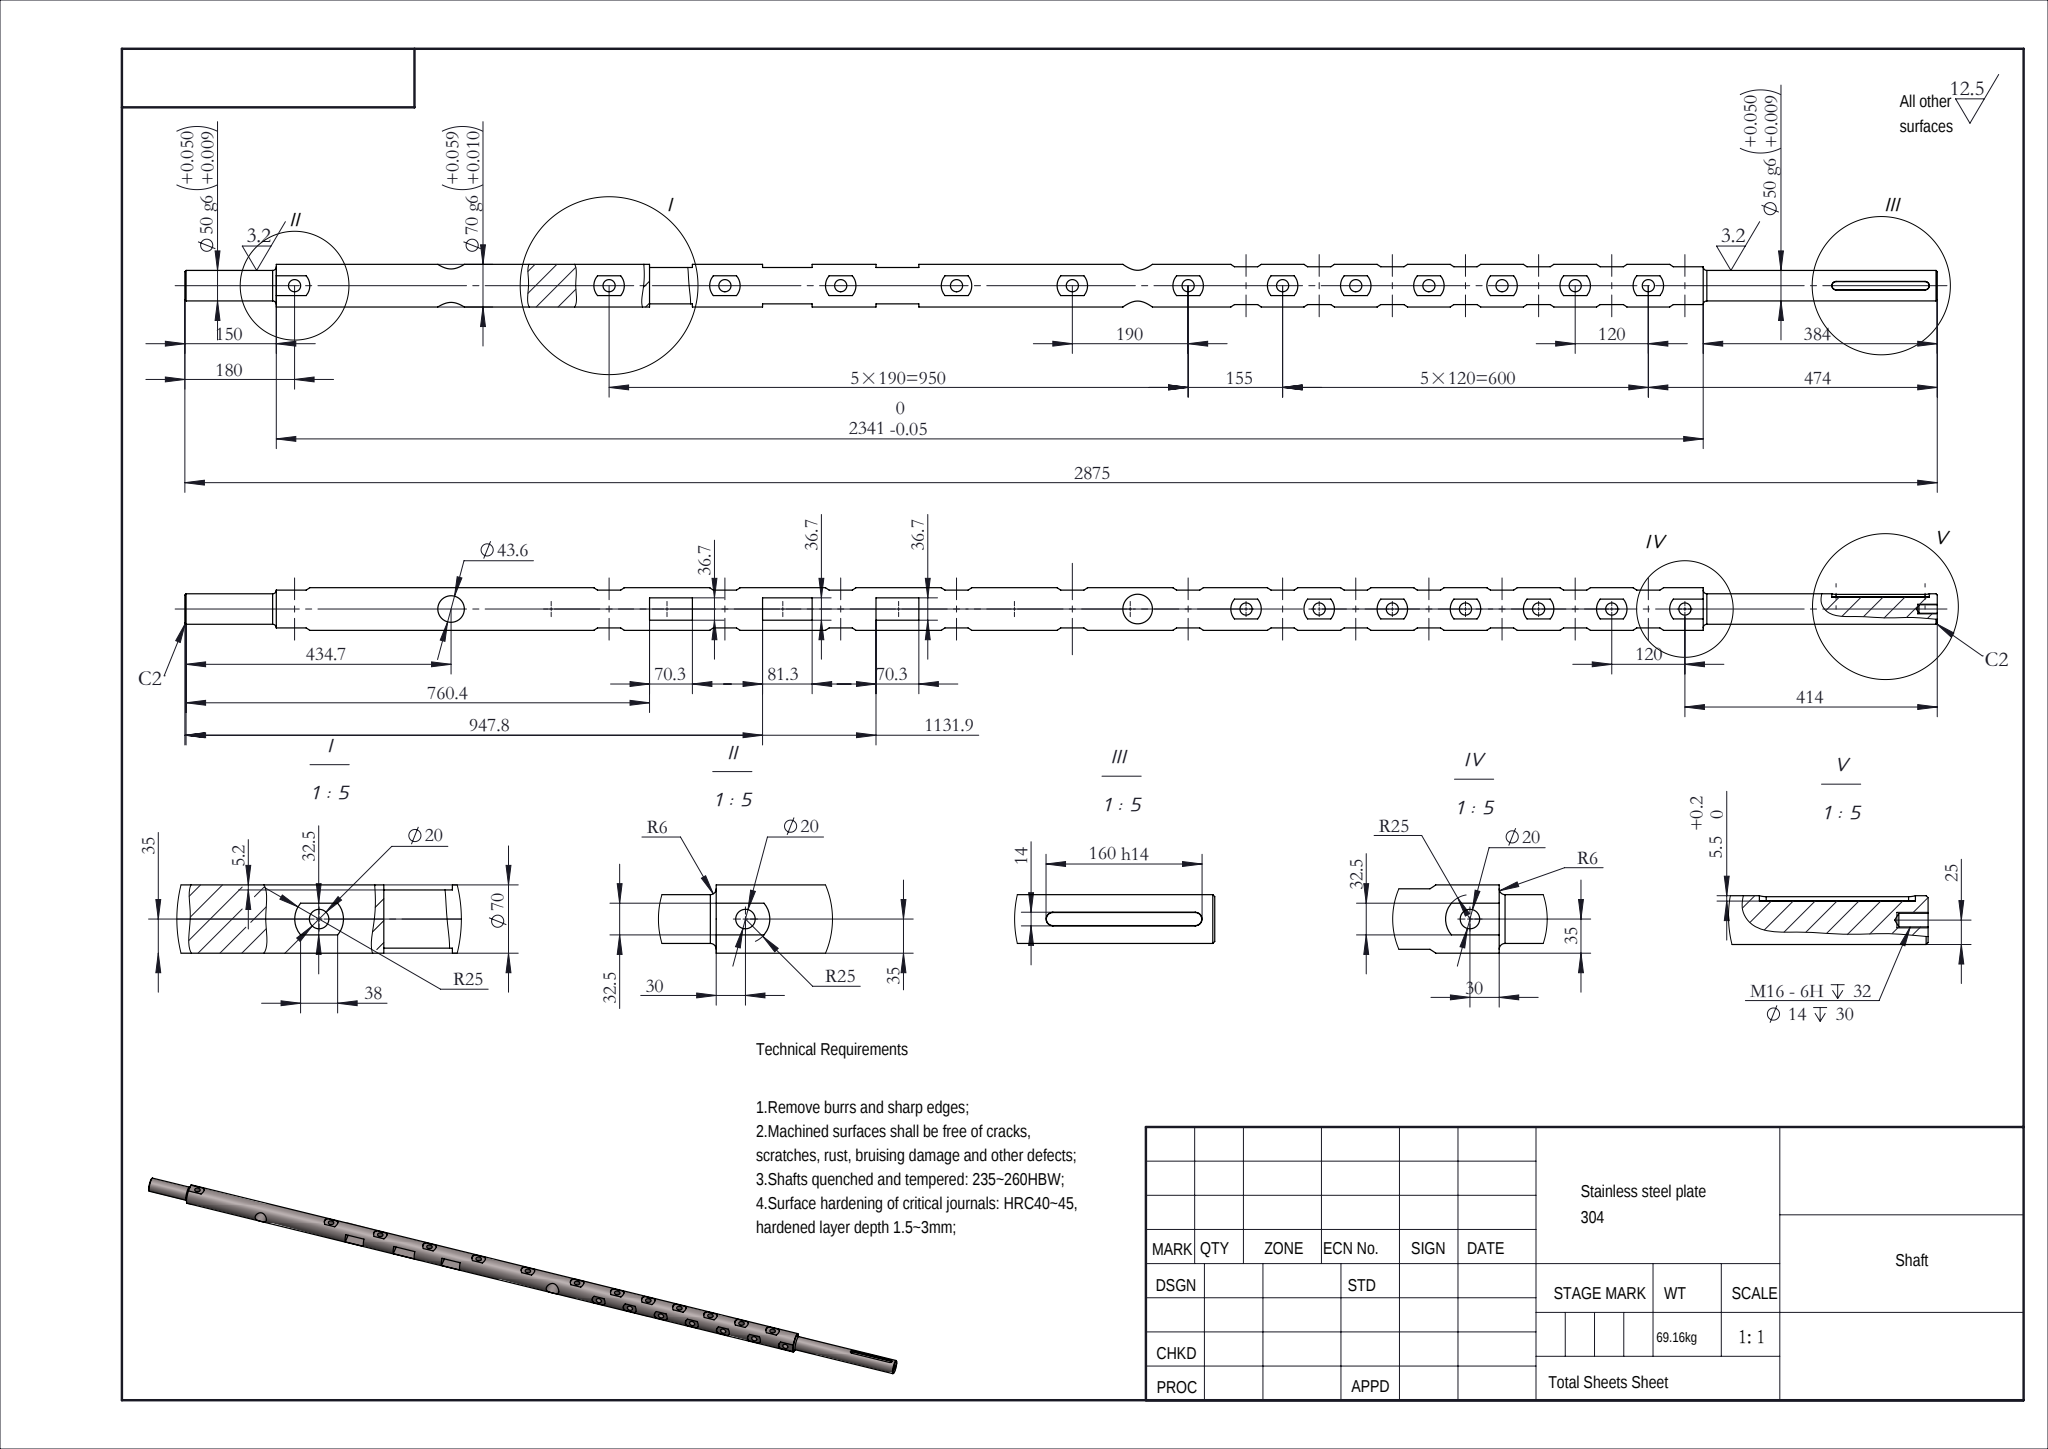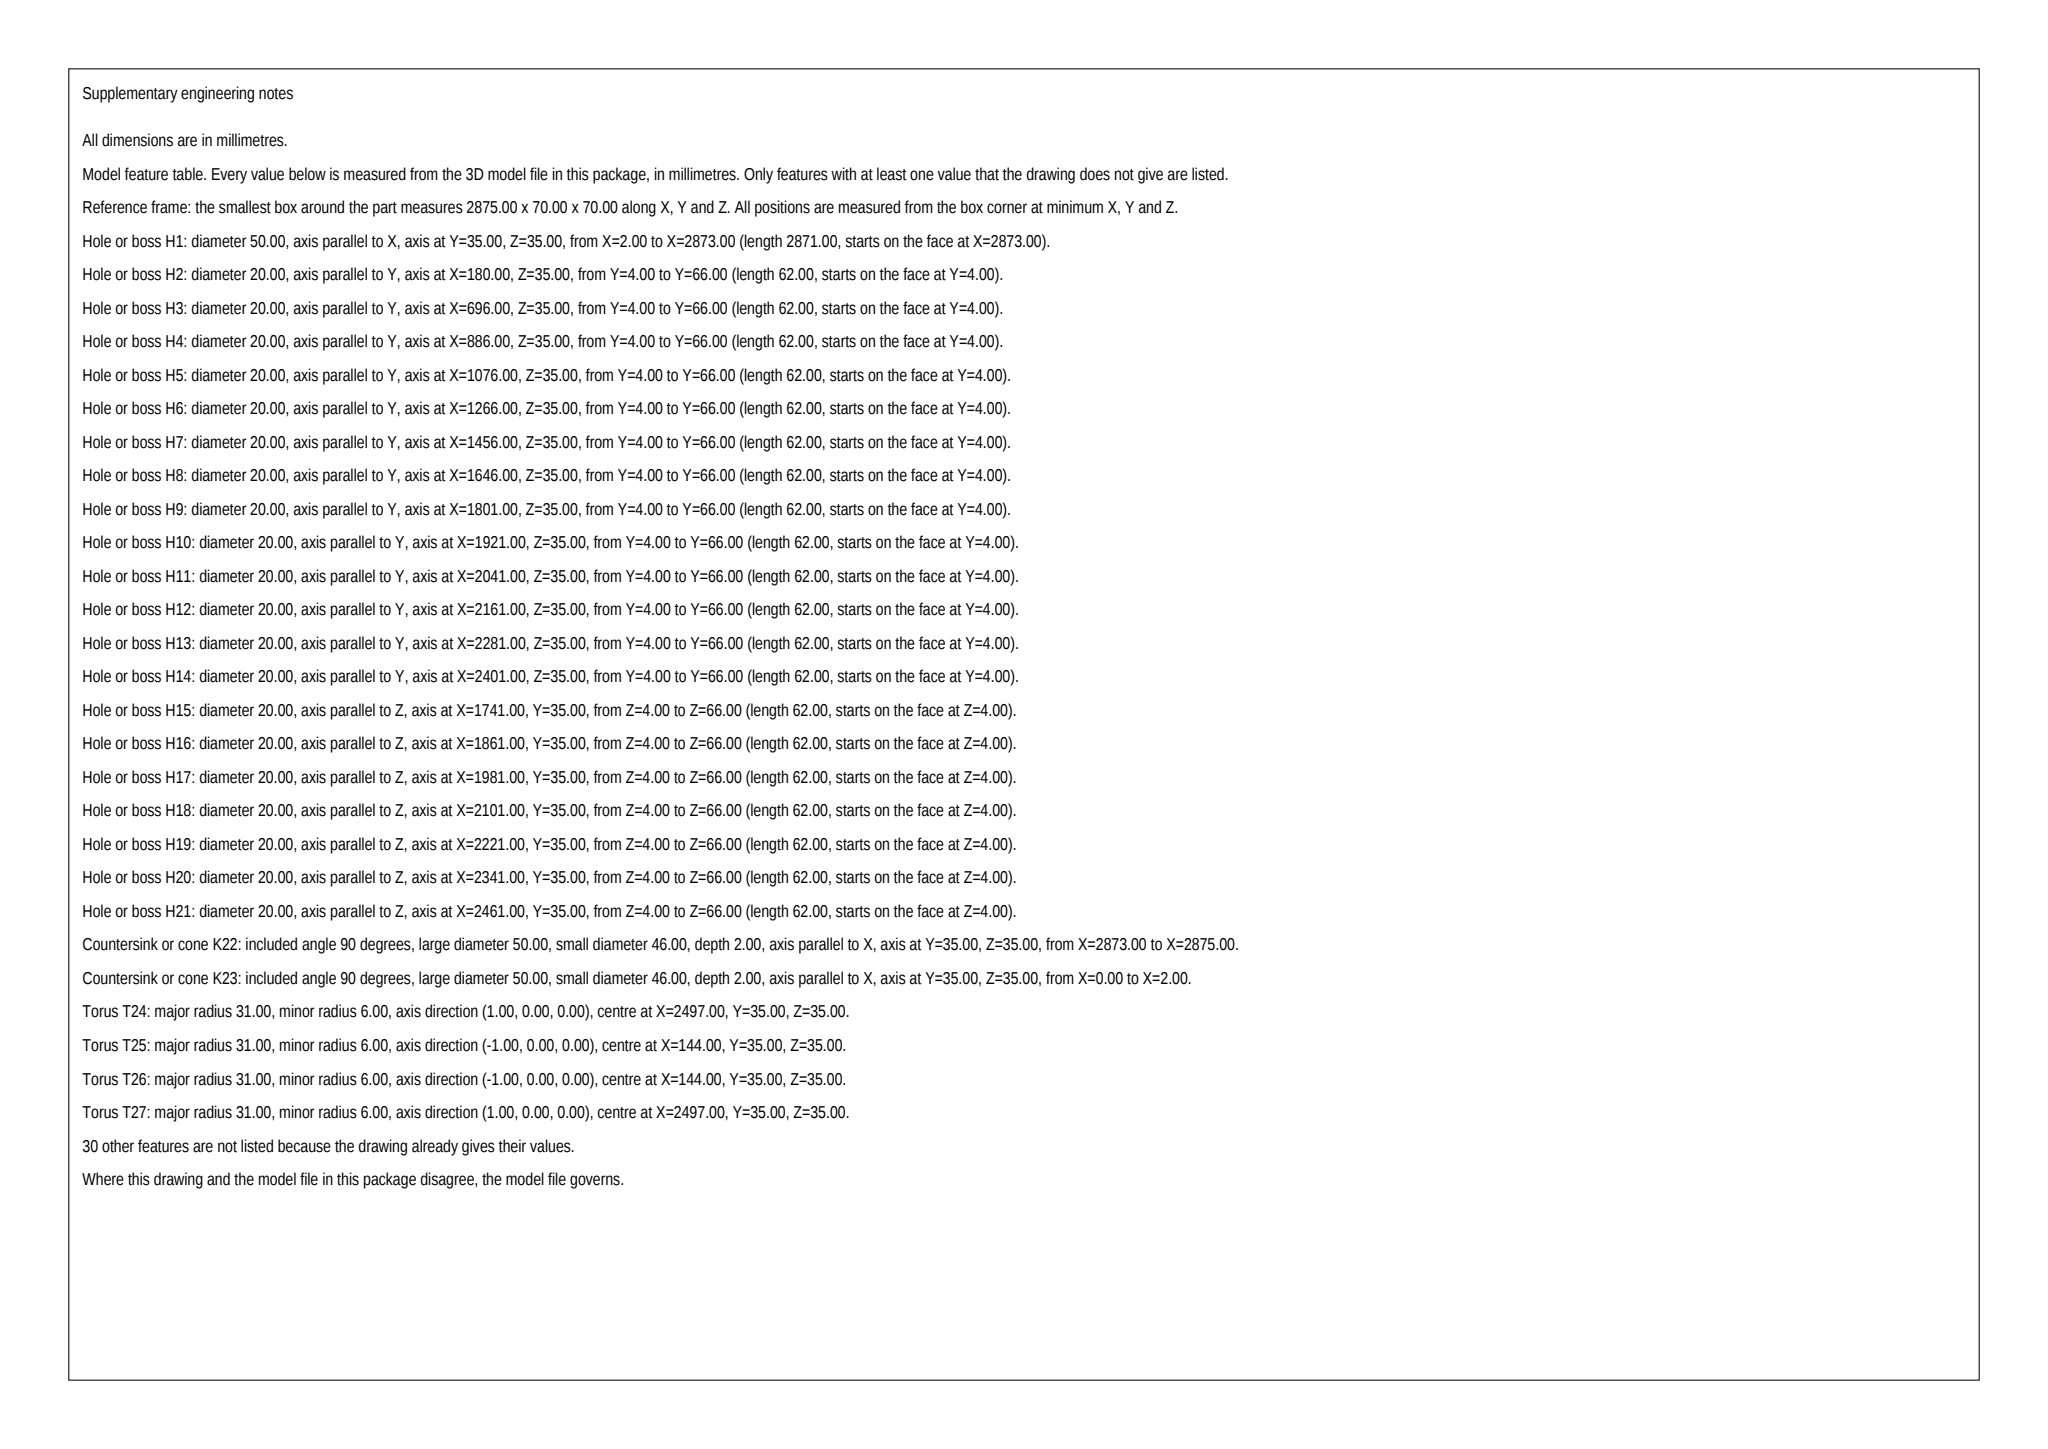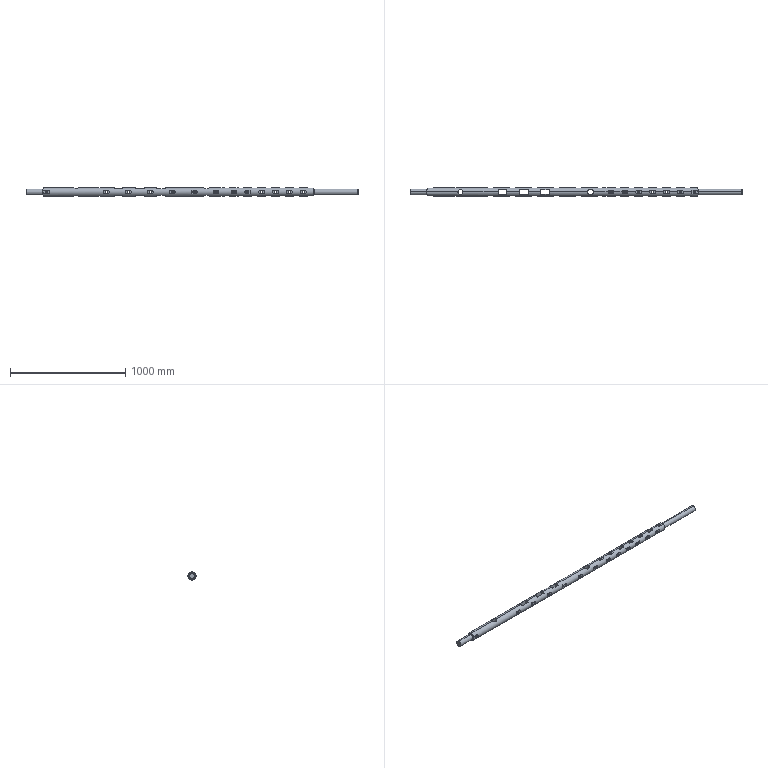Part | SolidWorks | mm | material Stainless steel plate 304 | 1 solid | 218 faces | box 2875 x 70 x 70 mm | volume 8721652 mm3 | cylinder 145 | plane 61 | cone 6 | torus 6 | commonest cylinder face diameters 50 x93 20 x40 14 x4 43.573 x2 48.573 x2 70 x2 0.6 x2